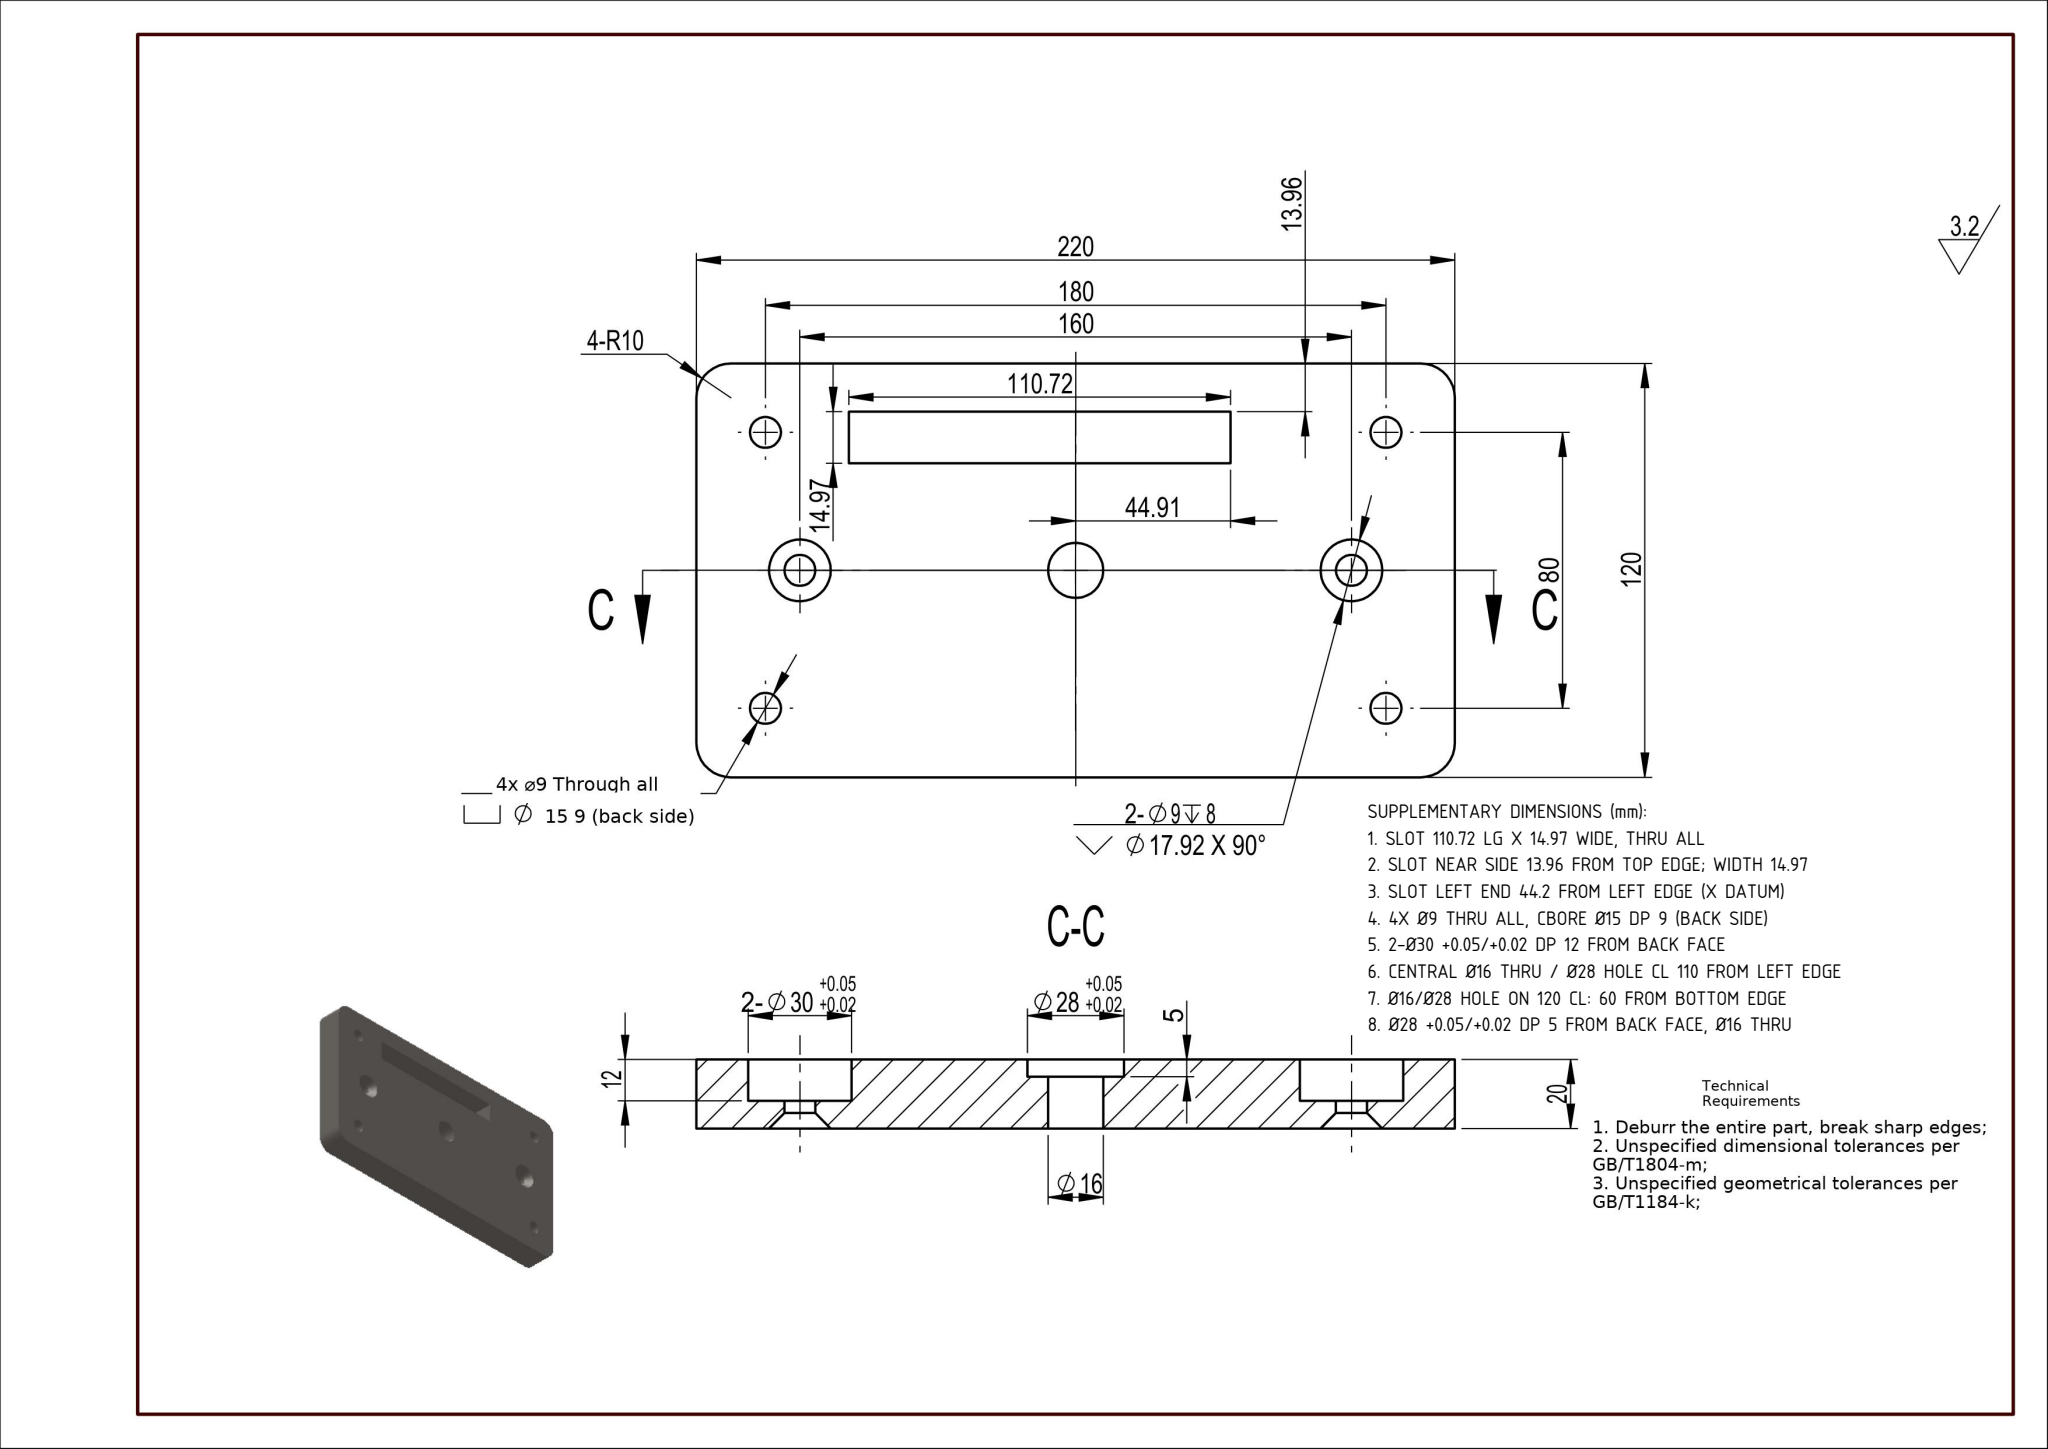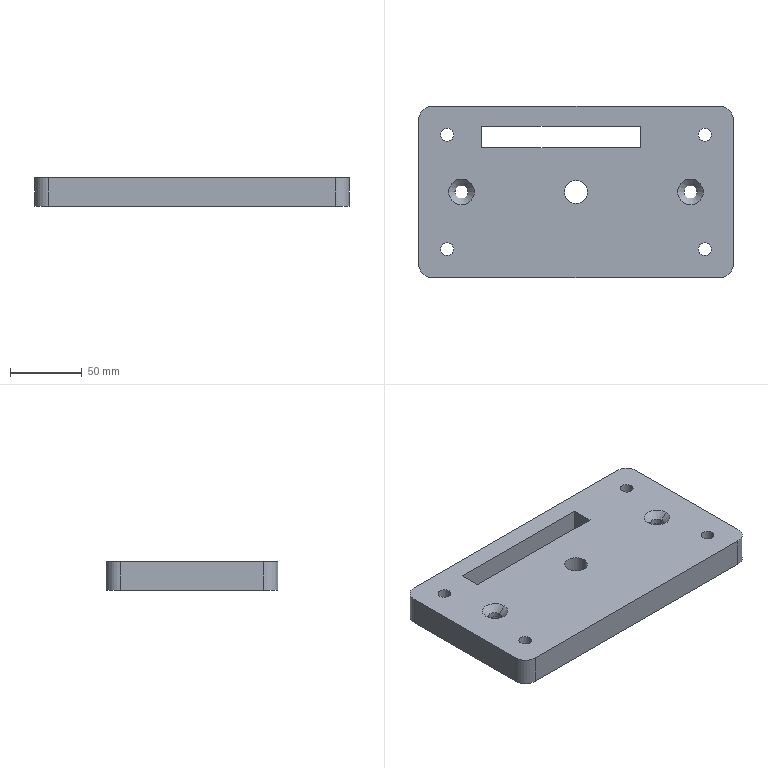Part | SolidWorks | mm | 1 solid | 53 faces | box 220 x 120 x 20 mm | volume 459147 mm3 | cylinder 32 | plane 17 | cone 4 | commonest cylinder face diameters 9 x12 15 x8 30 x4 20 x4 16 x2 28 x2
build123d program:
from build123d import *

# Parameters (mm, degrees)
SKETCH1_W                                            = 220
SKETCH1_H                                            = 120
EXTRUDE1_DEPTH                                       = 10
COUNTERSUNK_HOLE_FOR_M8_HEXAGONAL_COUNTE_D           = 9
COUNTERSUNK_HOLE_FOR_M8_HEXAGONAL_COUNTE_CSINK_D     = 17.92
COUNTERSUNK_HOLE_FOR_M8_HEXAGONAL_COUNTE_CSINK_ANGLE = 90
SKETCH5_R                                            = 15
CUT_EXTRUDE1_DEPTH                                   = 12
SKETCH8_R                                            = 14
CUT_EXTRUDE7_DEPTH                                   = 5
SKETCH15_R                                           = 8
CUT_EXTRUDE11_DEPTH                                  = 127.886
HOLE_SIZE_ACCORDING_TO_THE_TYPE_OF_HEX_S_D           = 9
HOLE_SIZE_ACCORDING_TO_THE_TYPE_OF_HEX_S_CBORE_D     = 15
HOLE_SIZE_ACCORDING_TO_THE_TYPE_OF_HEX_S_CBORE_DEPTH = 9
FILLET1_R                                            = 10
SKETCH18_W                                           = 110.715
SKETCH18_H                                           = 14.971
CUT_EXTRUDE12_DEPTH                                  = 92


with BuildPart() as part:
    # Sketch1 → Extrude1 (new, symmetric)
    with BuildSketch(Plane.XY):
        Rectangle(SKETCH1_W, SKETCH1_H)
    extrude(amount=EXTRUDE1_DEPTH, both=True)

    # Countersunk Hole for M8 Hexagonal Counte (through all)
    with Locations(Plane.XY.offset(10)):
        with Locations((-80, 0), (80, 0)):
            CounterSinkHole(COUNTERSUNK_HOLE_FOR_M8_HEXAGONAL_COUNTE_D / 2, COUNTERSUNK_HOLE_FOR_M8_HEXAGONAL_COUNTE_CSINK_D / 2, counter_sink_angle=COUNTERSUNK_HOLE_FOR_M8_HEXAGONAL_COUNTE_CSINK_ANGLE)

    # Sketch5 → Cut-Extrude1 (cut)
    with BuildSketch(Plane(origin=(0, 0, -10), x_dir=(-1, 0, 0), z_dir=(0, 0, -1))):
        with Locations((-80, 0)):
            Circle(SKETCH5_R)
        with Locations((80, 0)):
            Circle(SKETCH5_R)
    extrude(amount=-CUT_EXTRUDE1_DEPTH, mode=Mode.SUBTRACT)

    # Sketch8 → Cut-Extrude7 (cut)
    with BuildSketch(Plane.XY.offset(-10)):
        Circle(SKETCH8_R)
    extrude(amount=CUT_EXTRUDE7_DEPTH, mode=Mode.SUBTRACT)

    # Sketch15 → Cut-Extrude11 (cut, through all)
    with BuildSketch(Plane(origin=(0, 0, -10), x_dir=(-1, 0, 0), z_dir=(0, 0, -1))):
        Circle(SKETCH15_R)
    extrude(amount=-CUT_EXTRUDE11_DEPTH, mode=Mode.SUBTRACT)

    # Hole Size according to the type of Hex S (through all)
    with Locations(Plane(origin=(0, 0, -10), x_dir=(-1, 0, 0), z_dir=(0, 0, -1))):
        with Locations((-90, 40), (-90, -40), (90, -40), (90, 40)):
            CounterBoreHole(HOLE_SIZE_ACCORDING_TO_THE_TYPE_OF_HEX_S_D / 2, HOLE_SIZE_ACCORDING_TO_THE_TYPE_OF_HEX_S_CBORE_D / 2, HOLE_SIZE_ACCORDING_TO_THE_TYPE_OF_HEX_S_CBORE_DEPTH)

    # Fillet1
    fillet1_edges = [part.edges().sort_by_distance(p)[0] for p in [
        (-110, -60, 0),
        (-110, 60, 0),
        (110, 60, 0),
        (110, -60, 0),
    ]]
    fillet(fillet1_edges, radius=FILLET1_R)

    # Sketch18 → Cut-Extrude12 (cut)
    with BuildSketch(Plane(origin=(0, 0, -10), x_dir=(-1, 0, 0), z_dir=(0, 0, -1))):
        with Locations((10.445, 38.559)):
            Rectangle(SKETCH18_W, SKETCH18_H)
    extrude(amount=-CUT_EXTRUDE12_DEPTH, mode=Mode.SUBTRACT)


solid = part.part